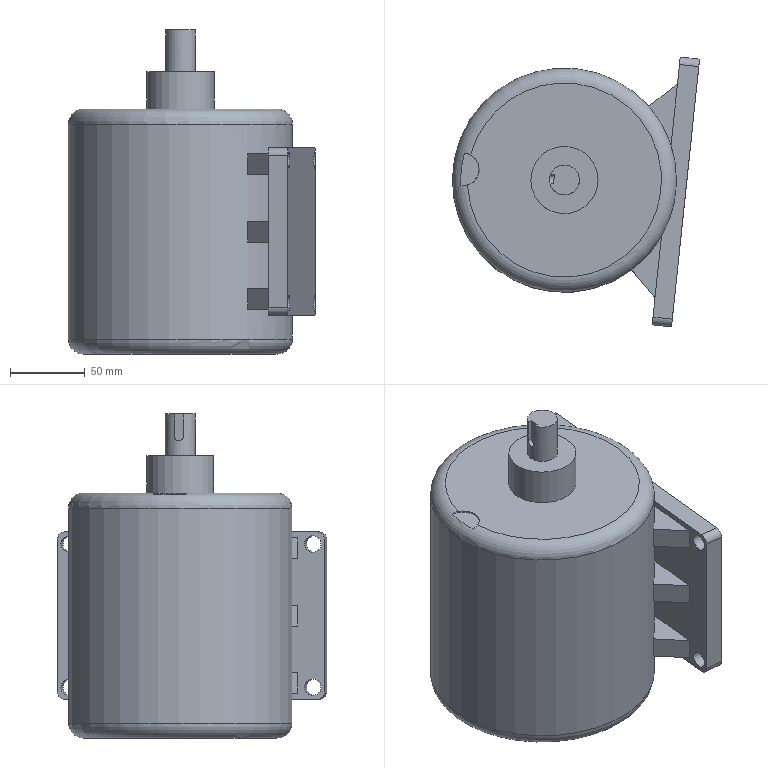Component | NX | MOTOR | 1 solid | 51 faces | volume 1002509 mm3 | plane 35 | cylinder 14 | torus 2 | commonest cylinder face diameters 11 x4 10 x4 150 x1 45 x1 20 x1 6 x1 22 x1 136 x1